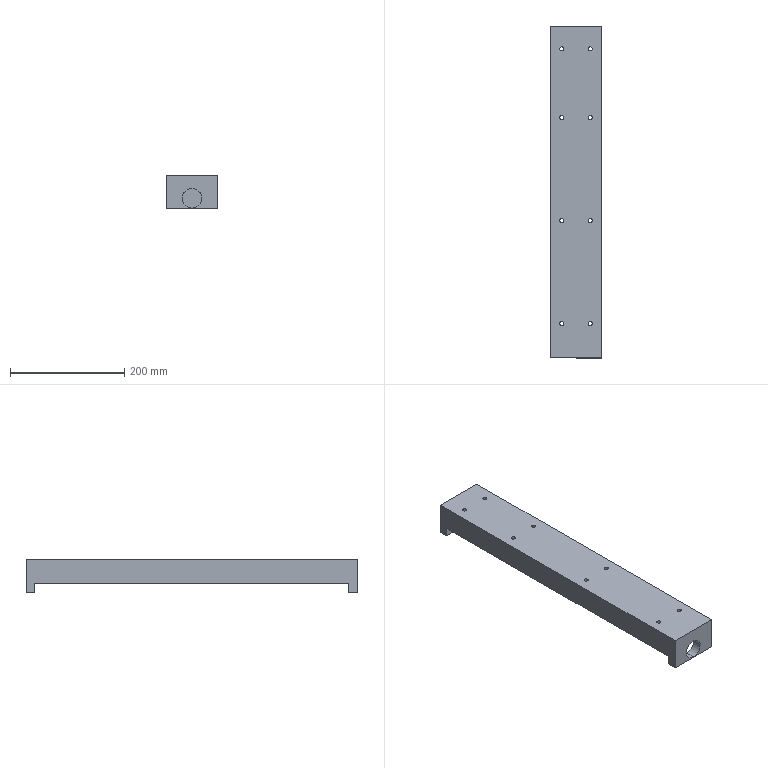Component | SolidWorks | Y-AxisAssembly-1_Y-AxisSlide-1 | 1 solid | 33 faces | box 90 x 580 x 58 mm | volume 1168912 mm3 | cylinder 18 | plane 15 | commonest cylinder face diameters 7 x16 34 x2